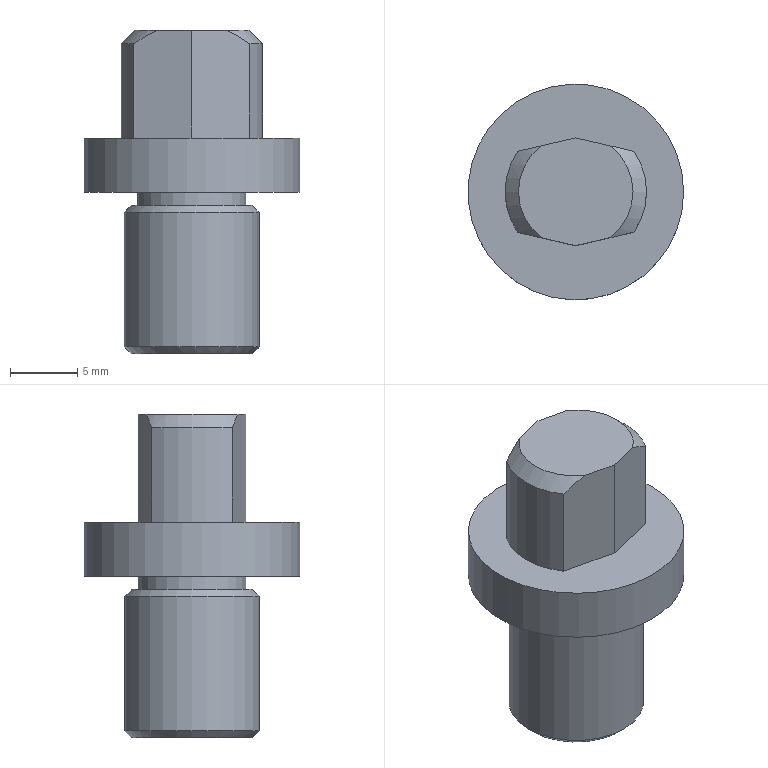Component | NX | B_LOC_PIN | 1 solid | 18 faces | volume 2248 mm3 | plane 9 | cylinder 5 | cone 4 | commonest cylinder face diameters 10.5 x2 10 x1 8 x1 16 x1